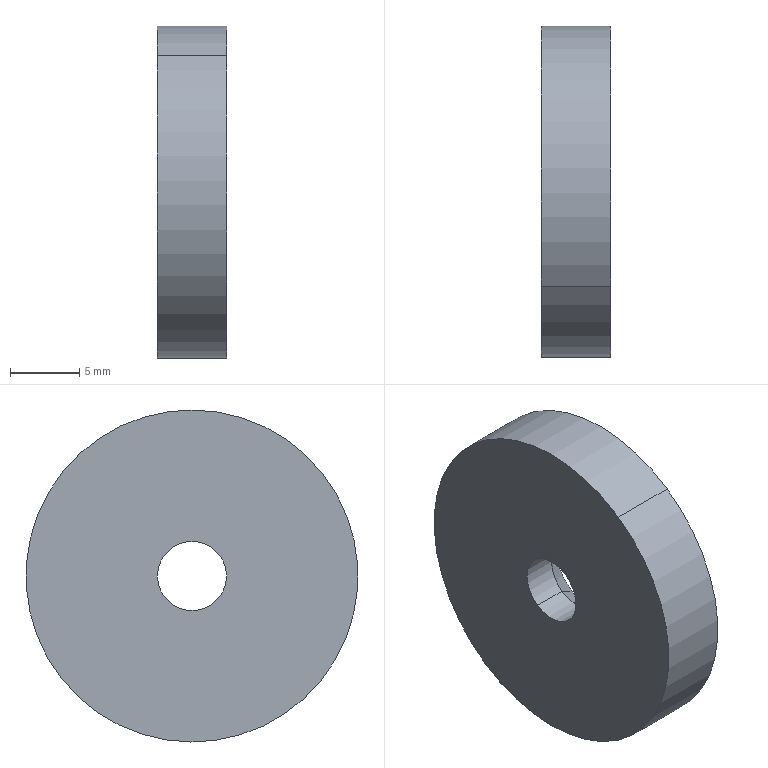Component | SolidWorks | Pillar-BeamConnectionGasket-2 | 1 solid | 8 faces | box 5 x 24 x 24 mm | volume 2098 mm3 | cylinder 4 | cone 2 | plane 2 | commonest cylinder face diameters 5 x2 24 x2
build123d program:
from build123d import *

# Parameters (mm, degrees)
SKETCH1_R           = 12
BOSS_EXTRUDE1_DEPTH = 5
SKETCH2_R           = 2.5
CUT_EXTRUDE1_DEPTH  = 18.692
CHAMFER1_SIZE       = 2.5


with BuildPart() as part:
    # Sketch1 → Boss-Extrude1 (new body)
    with BuildSketch(Plane.XY):
        Circle(SKETCH1_R)
    extrude(amount=BOSS_EXTRUDE1_DEPTH)

    # Sketch2 → Cut-Extrude1 (cut, through all)
    with BuildSketch(Plane.XY.offset(5)):
        Circle(SKETCH2_R)
    extrude(amount=-CUT_EXTRUDE1_DEPTH, mode=Mode.SUBTRACT)

    # Chamfer1
    chamfer1_edges = [part.edges().sort_by_distance(p)[0] for p in [
        (-2.5, 0, 5),
    ]]
    chamfer(chamfer1_edges, length=CHAMFER1_SIZE)


solid = part.part

# Placed as in the assembly
solid = solid.moved(Location((-34.428, 27.796, 284.382), (0, 90, 0)))